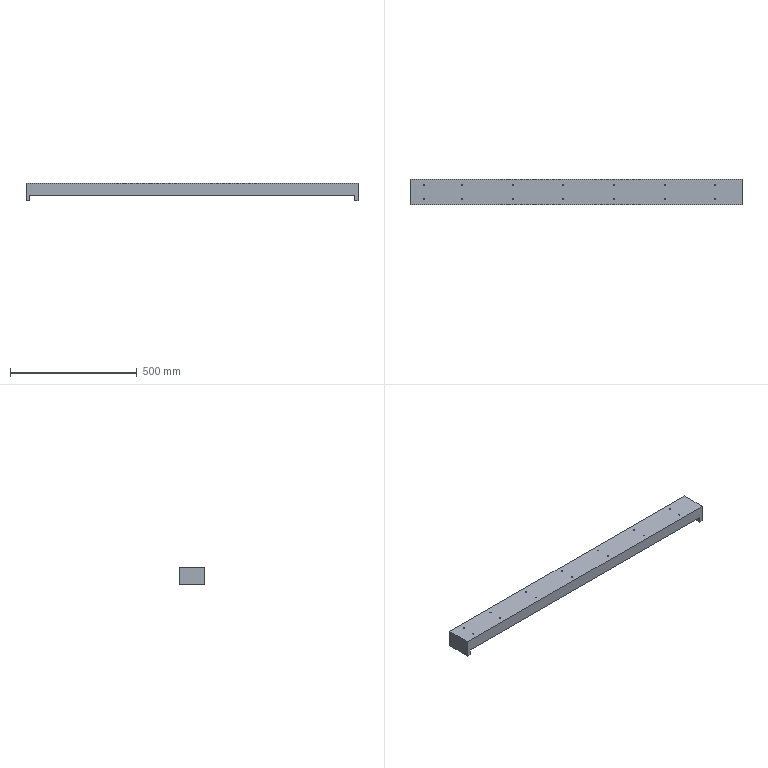Component | SolidWorks | X-AxisSlide-1 | 1 solid | 44 faces | box 1310 x 100 x 69 mm | volume 2895258 mm3 | cylinder 30 | plane 14 | commonest cylinder face diameters 4.2 x28 30 x2
build123d program:
from build123d import *

# Parameters (mm, degrees)
SKETCH1_W                  = 1310
SKETCH1_H                  = 100
BOSS_EXTRUDE1_DEPTH        = 69
SKETCH2_W                  = 1280
SKETCH2_H                  = 70
CUT_EXTRUDE1_DEPTH         = 59
SKETCH3_W                  = 1280
SKETCH3_H                  = 164.096
CUT_EXTRUDE2_DEPTH         = 22
SKETCH4_R                  = 15
CUT_EXTRUDE3_DEPTH         = 22
M5_TAPPED_HOLE1_AT_2_COUNT = 2
M5_TAPPED_HOLE1_AT_2_PITCH = 54
LPATTERN1_COUNT            = 6
LPATTERN1_PITCH            = 200
M5_TAPPED_HOLE2_D          = 4.2
M5_TAPPED_HOLE2_DEPTH      = 12.4
M5_TAPPED_HOLE2_TIP        = 1.262


with BuildPart() as part:
    # Sketch1 → Boss-Extrude1 (new body)
    with BuildSketch(Plane.XY):
        Rectangle(SKETCH1_W, SKETCH1_H)
    extrude(amount=BOSS_EXTRUDE1_DEPTH)

    # Sketch2 → Cut-Extrude1 (cut)
    with BuildSketch(Plane.XY):
        Rectangle(SKETCH2_W, SKETCH2_H)
    extrude(amount=CUT_EXTRUDE1_DEPTH, mode=Mode.SUBTRACT)

    # Sketch3 → Cut-Extrude2 (cut)
    with BuildSketch(Plane.XY):
        with Locations((0, -32.048)):
            Rectangle(SKETCH3_W, SKETCH3_H)
    extrude(amount=CUT_EXTRUDE2_DEPTH, mode=Mode.SUBTRACT)

    # Sketch4 → Cut-Extrude3 (cut)
    with BuildSketch(Plane(origin=(655, 0, 0), x_dir=(0, 0, -1), z_dir=(1, 0, 0))):
        with Locations((-29, 0)):
            Circle(SKETCH4_R)
    extrude(amount=-CUT_EXTRUDE3_DEPTH, mode=Mode.SUBTRACT)

    # Sketch5 → M5 Tapped Hole1 (revolve, cut)
    with BuildSketch(Plane(origin=(550, 27, 69), x_dir=(0, -1, 0), z_dir=(1, 0, 0))):
        Polygon((0, 0), (0, 13.662), (2.1, 12.4), (2.1, 0), align=None)
    m5_tapped_hole1 = revolve(axis=Axis((550, 27, 75.35), (0, 0, -1)), mode=Mode.SUBTRACT)

    # M5 Tapped Hole1 at 2: M5 Tapped Hole1 ×2
    with Locations(*[(0, -i * M5_TAPPED_HOLE1_AT_2_PITCH, 0) for i in range(1, M5_TAPPED_HOLE1_AT_2_COUNT)]):
        add(m5_tapped_hole1, mode=Mode.SUBTRACT)

    # LPattern1: M5 Tapped Hole1 ×6
    with Locations(*[(-i * LPATTERN1_PITCH, 0, 0) for i in range(1, LPATTERN1_COUNT)]):
        add(m5_tapped_hole1, mode=Mode.SUBTRACT)

    # LPattern1 copy 1 sketch → LPattern1 copy 1 (revolve, cut)
    with BuildSketch(Plane(origin=(350, -27, 69), x_dir=(0, -1, 0), z_dir=(1, 0, 0))):
        Polygon((0, 0), (0, 13.662), (2.1, 12.4), (2.1, 0), align=None)
    revolve(axis=Axis((350, -27, 75.35), (0, 0, -1)), mode=Mode.SUBTRACT)

    # LPattern1 copy 2 sketch → LPattern1 copy 2 (revolve, cut)
    with BuildSketch(Plane(origin=(150, -27, 69), x_dir=(0, -1, 0), z_dir=(1, 0, 0))):
        Polygon((0, 0), (0, 13.662), (2.1, 12.4), (2.1, 0), align=None)
    revolve(axis=Axis((150, -27, 75.35), (0, 0, -1)), mode=Mode.SUBTRACT)

    # LPattern1 copy 3 sketch → LPattern1 copy 3 (revolve, cut)
    with BuildSketch(Plane(origin=(-50, -27, 69), x_dir=(0, -1, 0), z_dir=(1, 0, 0))):
        Polygon((0, 0), (0, 13.662), (2.1, 12.4), (2.1, 0), align=None)
    revolve(axis=Axis((-50, -27, 75.35), (0, 0, -1)), mode=Mode.SUBTRACT)

    # LPattern1 copy 4 sketch → LPattern1 copy 4 (revolve, cut)
    with BuildSketch(Plane(origin=(-250, -27, 69), x_dir=(0, -1, 0), z_dir=(1, 0, 0))):
        Polygon((0, 0), (0, 13.662), (2.1, 12.4), (2.1, 0), align=None)
    revolve(axis=Axis((-250, -27, 75.35), (0, 0, -1)), mode=Mode.SUBTRACT)

    # LPattern1 copy 5 sketch → LPattern1 copy 5 (revolve, cut)
    with BuildSketch(Plane(origin=(-450, -27, 69), x_dir=(0, -1, 0), z_dir=(1, 0, 0))):
        Polygon((0, 0), (0, 13.662), (2.1, 12.4), (2.1, 0), align=None)
    revolve(axis=Axis((-450, -27, 75.35), (0, 0, -1)), mode=Mode.SUBTRACT)

    # M5 Tapped Hole2
    with Locations(Plane(origin=(-600, 27, 69), x_dir=(1, 0, 0), z_dir=(0, 0, 1))):
        with Locations((0, 0), (0, -54)):
            Hole(M5_TAPPED_HOLE2_D / 2, depth=M5_TAPPED_HOLE2_DEPTH)
            with Locations((0, 0, -(M5_TAPPED_HOLE2_DEPTH + M5_TAPPED_HOLE2_TIP / 2))):  # 118° drill point
                Cone(0, M5_TAPPED_HOLE2_D / 2, M5_TAPPED_HOLE2_TIP, mode=Mode.SUBTRACT)


solid = part.part